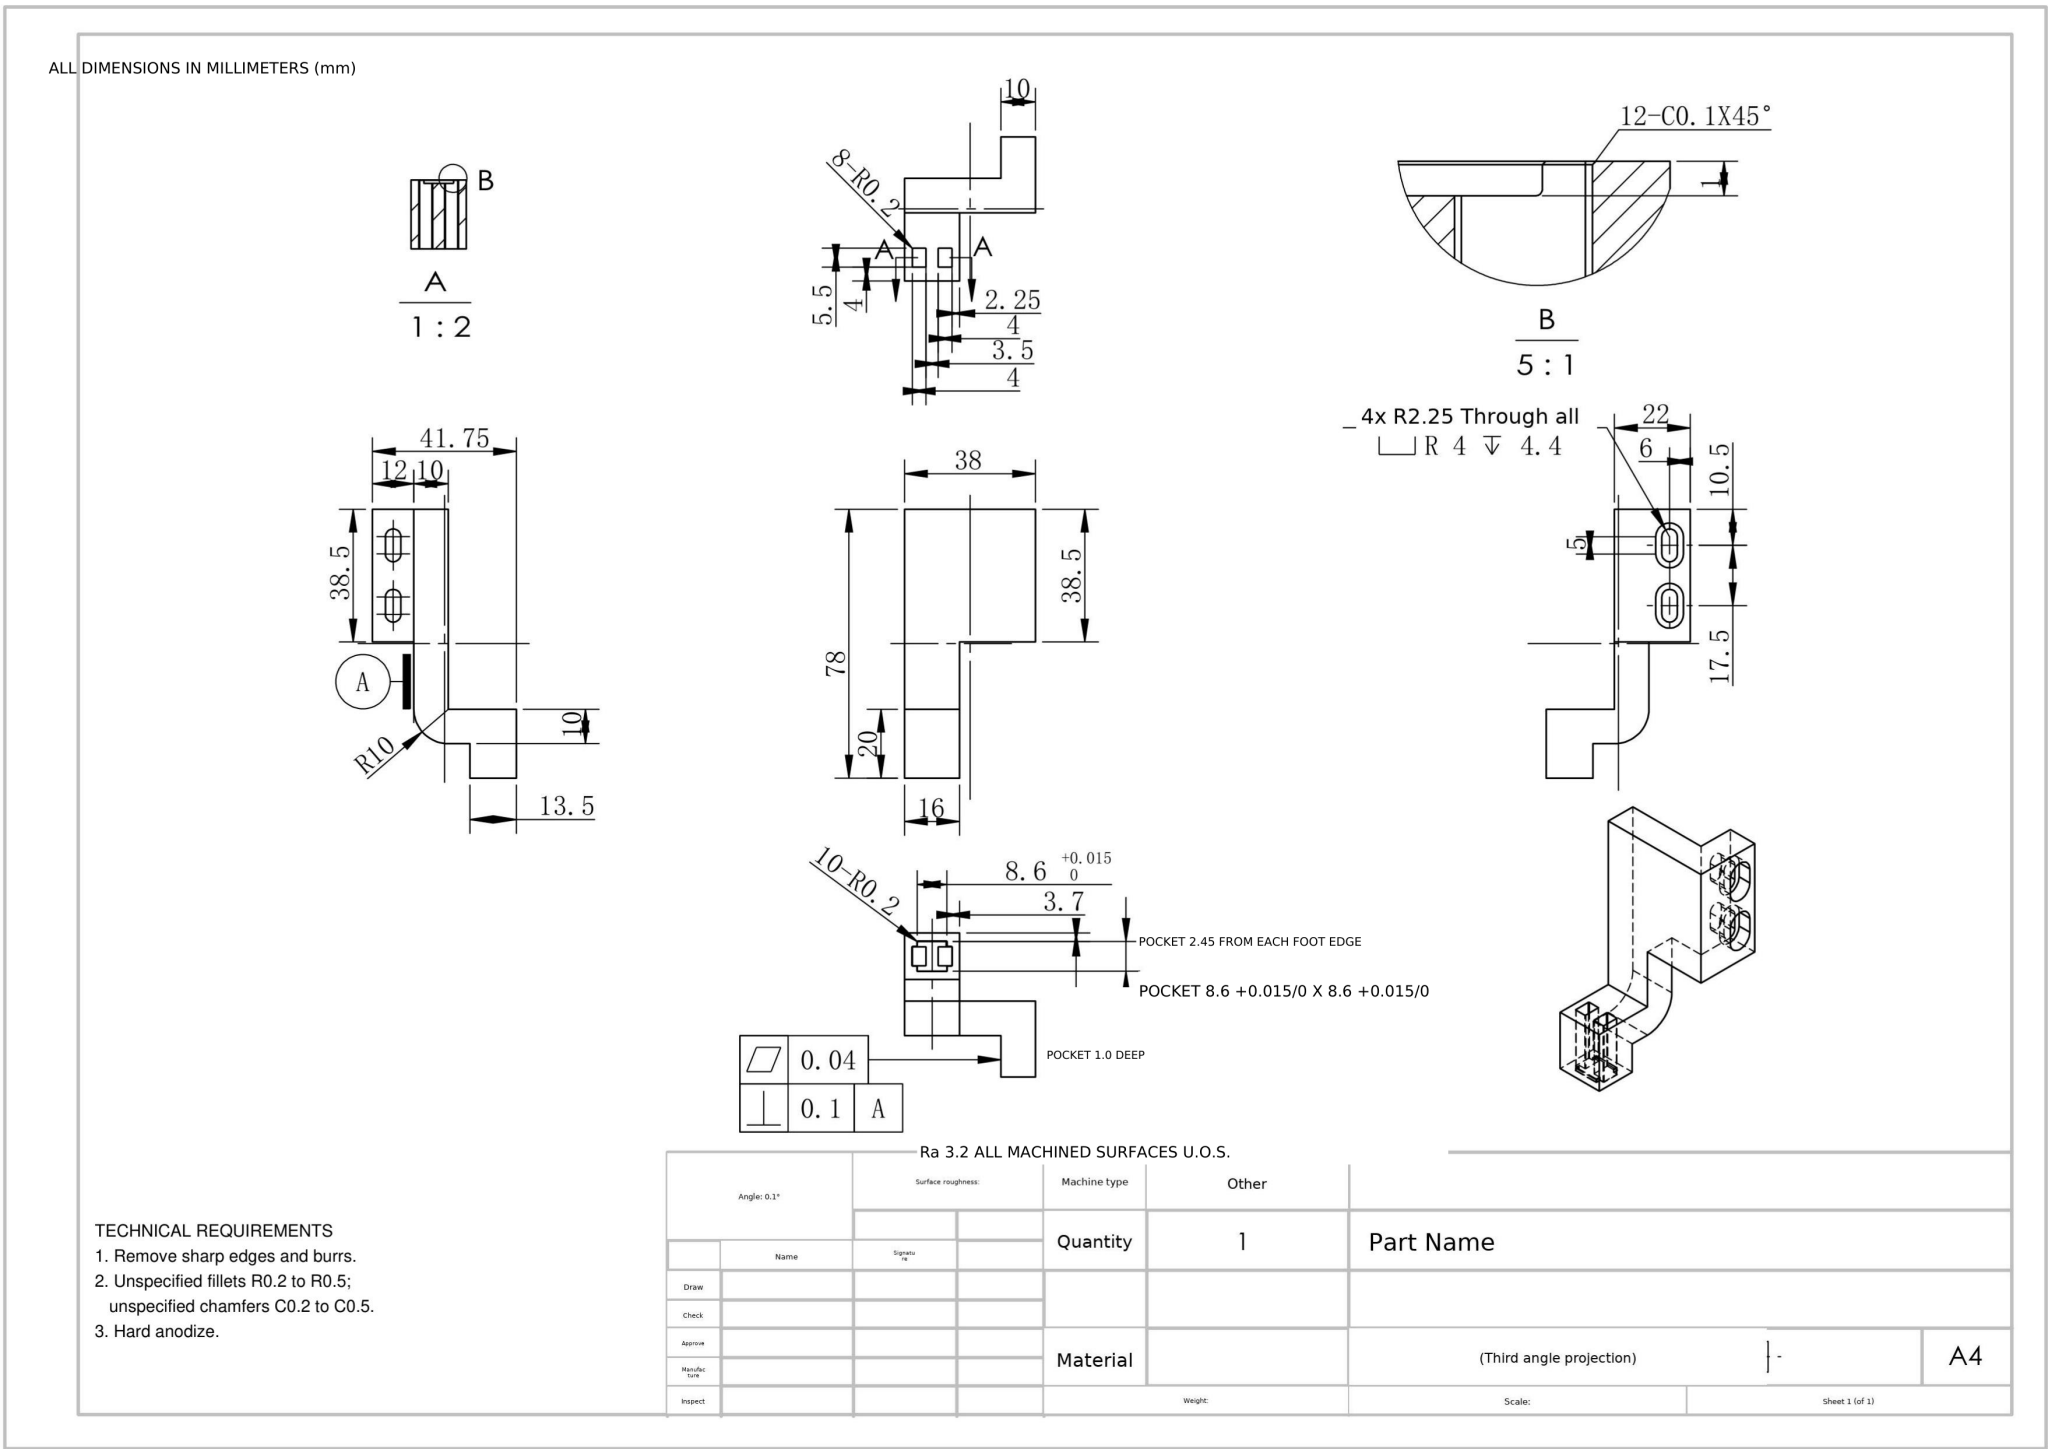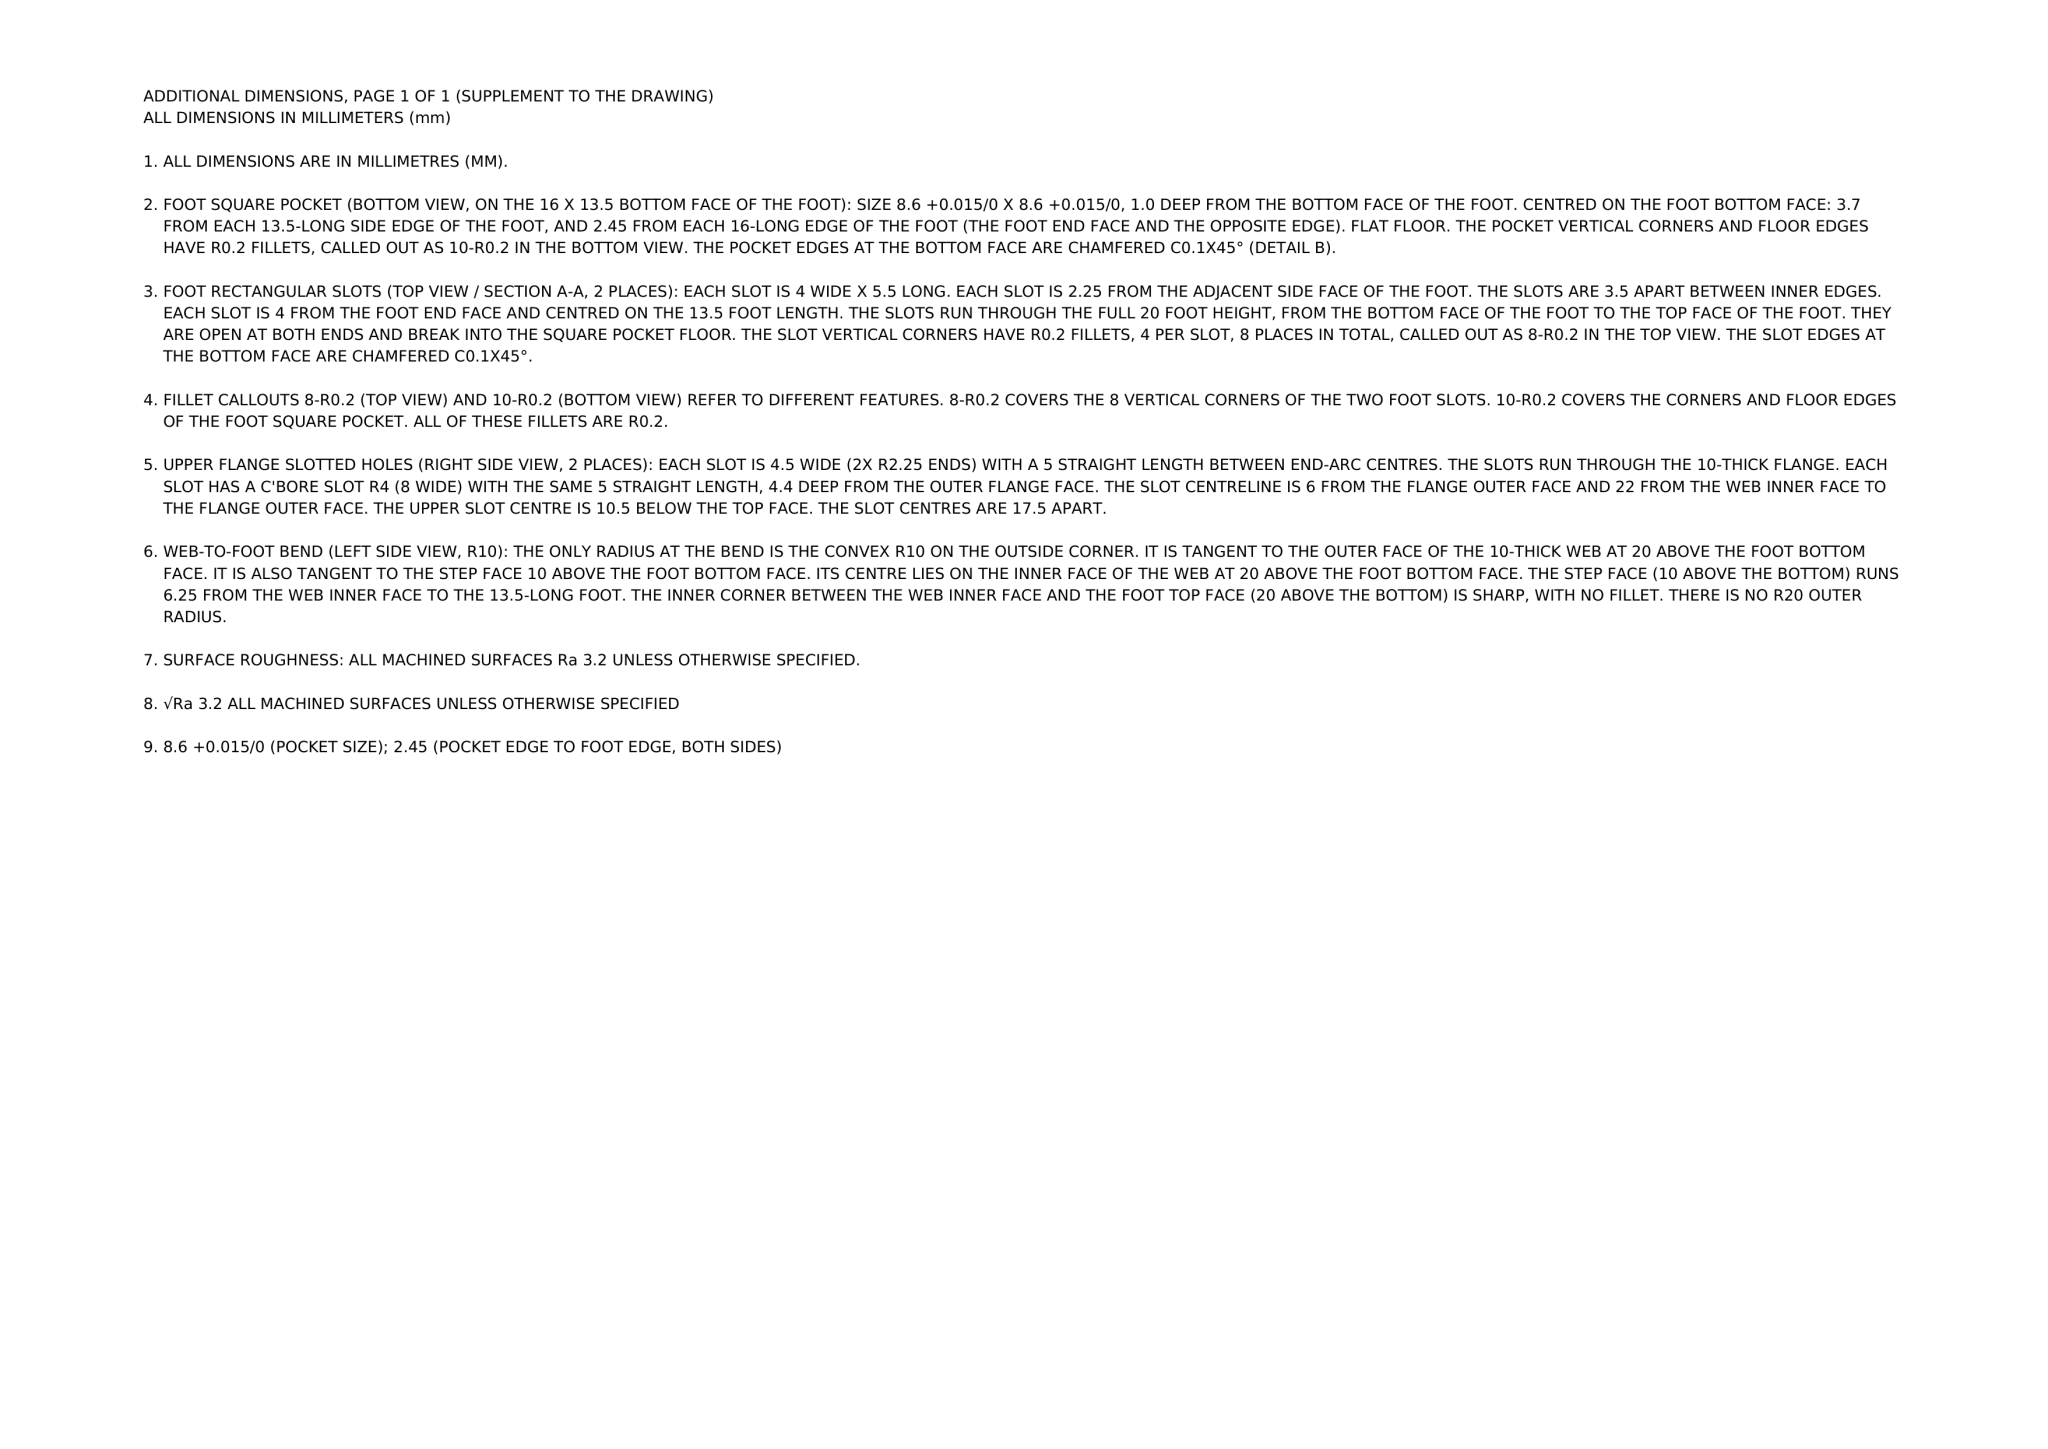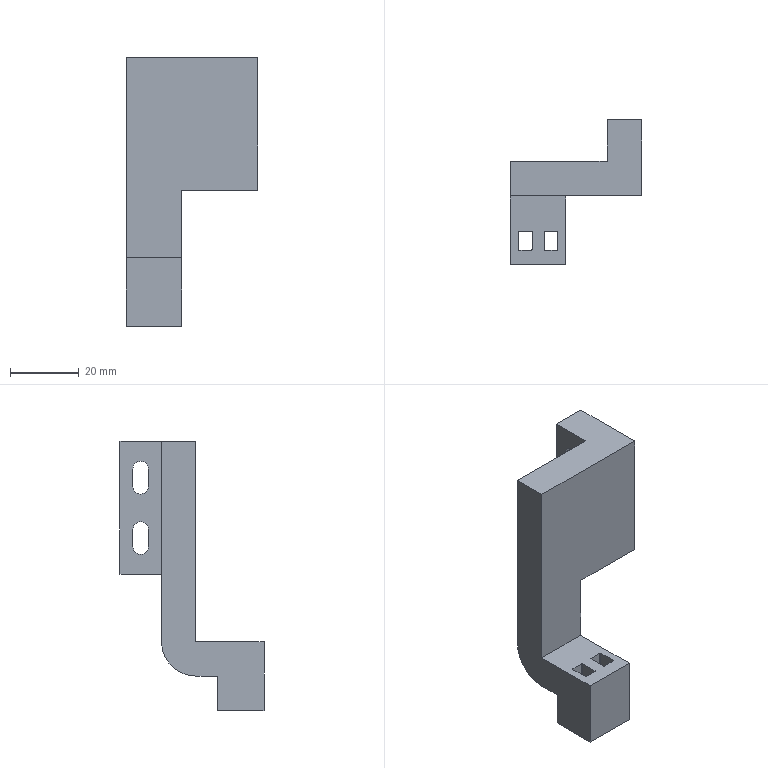Part | NX | mm | 1 solid | 94 faces | box 38 x 41.75 x 78 mm | volume 26798 mm3 | plane 51 | cylinder 31 | cone 8 | sphere 4 | commonest cylinder face diameters 0.4 x18 4.5 x6 8 x6 20 x1